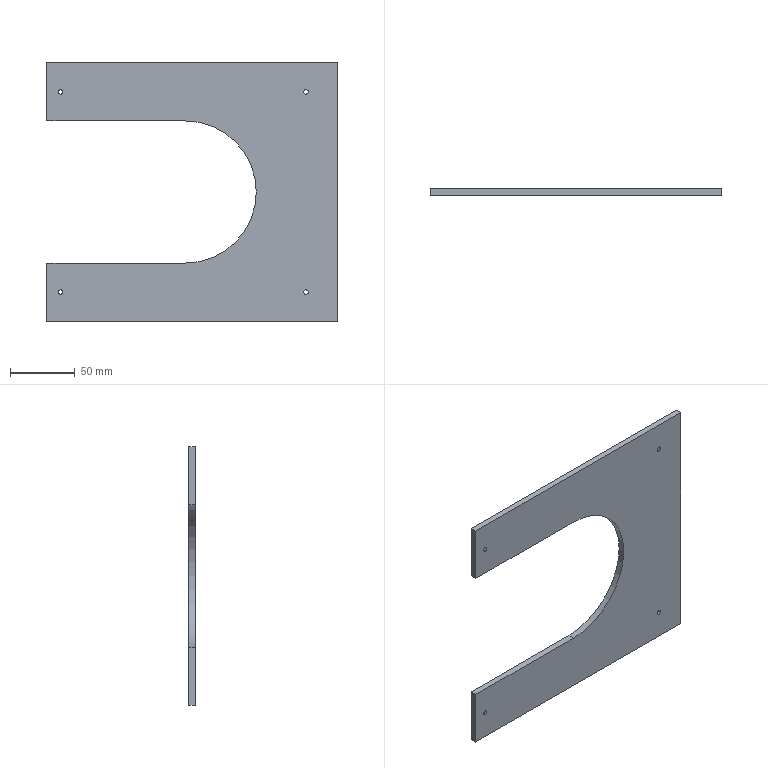CAM job | Mastercam | mm | 4 operations | part box 224.5 x 5 x 200
1. Contour (Ramp) | 3 - 3 平铣刀
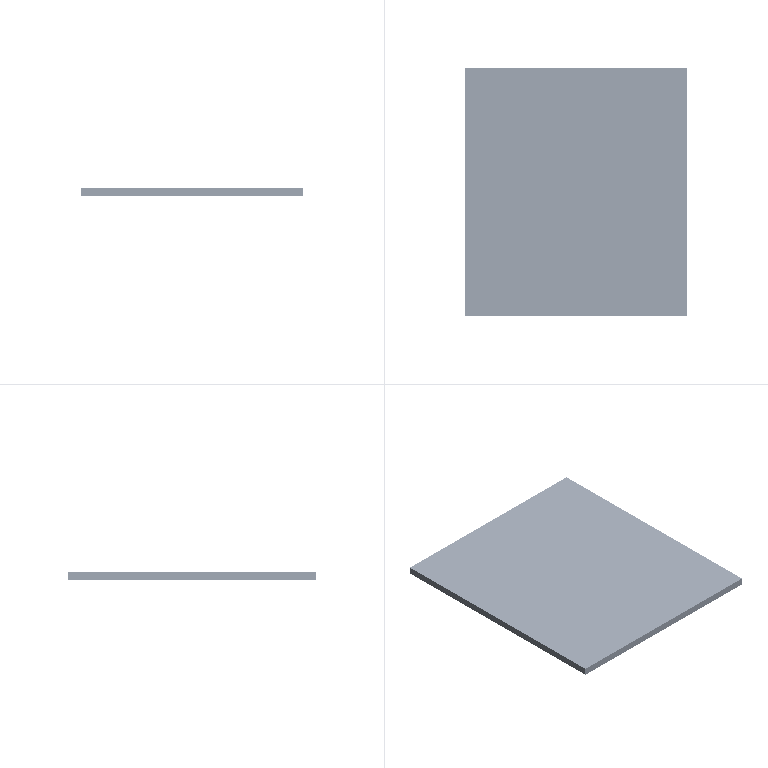2. Contour (2D) | 3 - 3 平铣刀
3. Contour (2D chamfer) | 7 - 4 倒角刀
4. Drill/Counterbore | 7 - 4 倒角刀